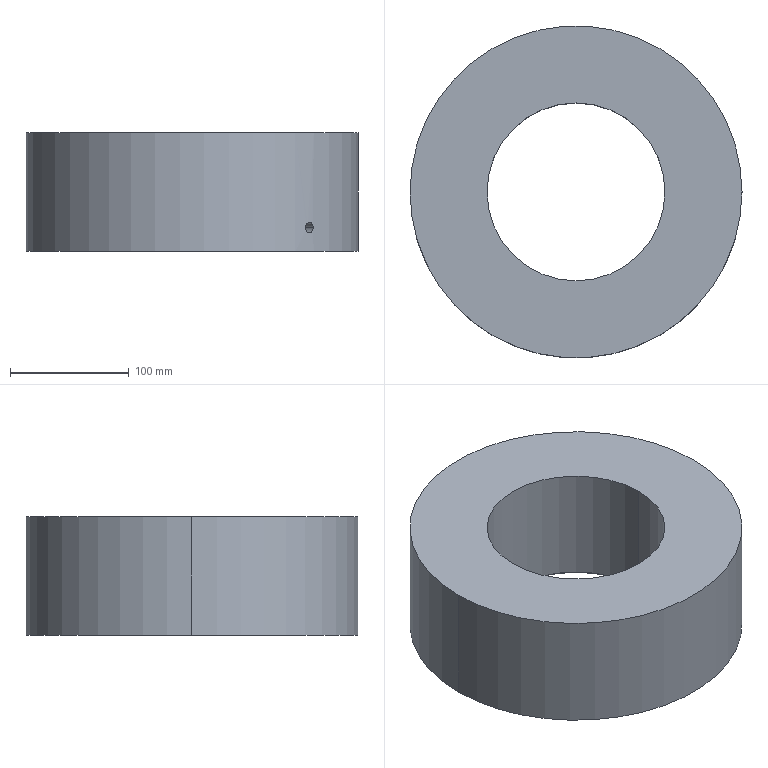Component | SolidWorks | JF21-80.1-1-3(_)-1-SOLID27-1 | 1 solid | 14 faces | box 280 x 280 x 100 mm | volume 4386913 mm3 | cylinder 8 | cone 4 | plane 2 | commonest cylinder face diameters 9 x2 7.5 x2 150 x2 280 x2
STEP:
#1=COLOUR_RGB('',0.7922,0.8196,0.9333);
#2=FILL_AREA_STYLE_COLOUR('',#1);
#3=FILL_AREA_STYLE('',(#2));
#4=SURFACE_STYLE_FILL_AREA(#3);
#5=SURFACE_SIDE_STYLE('',(#4));
#6=SURFACE_STYLE_USAGE(.BOTH.,#5);
#7=PRESENTATION_STYLE_ASSIGNMENT((#6));
#8=CARTESIAN_POINT('',(2.953,0.,7.323));
#9=VERTEX_POINT('',#8);
#10=CARTESIAN_POINT('',(-2.953,0.,7.323));
#11=VERTEX_POINT('',#10);
#12=CARTESIAN_POINT('',(0.,0.,7.323));
#13=DIRECTION('',(0.,0.,-1.));
#14=DIRECTION('',(1.,0.,0.));
#15=AXIS2_PLACEMENT_3D('',#12,#13,#14);
#16=CIRCLE('',#15,2.953);
#17=EDGE_CURVE('',#9,#11,#16,.T.);
#18=ORIENTED_EDGE('',*,*,#17,.F.);
#19=CARTESIAN_POINT('',(2.992,0.,7.283));
#20=VERTEX_POINT('',#19);
#21=CARTESIAN_POINT('',(2.992,0.,7.283));
#22=DIRECTION('',(-0.7071,-0.,0.7071));
#23=VECTOR('',#22,39.37);
#24=LINE('',#21,#23);
#25=EDGE_CURVE('',#20,#9,#24,.T.);
#26=ORIENTED_EDGE('',*,*,#25,.F.);
#27=CARTESIAN_POINT('',(-2.992,0.,7.283));
#28=VERTEX_POINT('',#27);
#29=CARTESIAN_POINT('',(0.,0.,7.283));
#30=DIRECTION('',(0.,0.,1.));
#31=DIRECTION('',(1.,0.,0.));
#32=AXIS2_PLACEMENT_3D('',#29,#30,#31);
#33=CIRCLE('',#32,2.992);
#34=EDGE_CURVE('',#28,#20,#33,.T.);
#35=ORIENTED_EDGE('',*,*,#34,.F.);
#36=CARTESIAN_POINT('',(-2.992,0.,7.283));
#37=DIRECTION('',(0.7071,0.,0.7071));
#38=VECTOR('',#37,39.37);
#39=LINE('',#36,#38);
#40=EDGE_CURVE('',#28,#11,#39,.T.);
#41=ORIENTED_EDGE('',*,*,#40,.T.);
#42=EDGE_LOOP('',(#18,#26,#35,#41));
#43=FACE_OUTER_BOUND('',#42,.T.);
#44=CARTESIAN_POINT('',(0.,0.,7.283));
#45=DIRECTION('',(0.,0.,-1.));
#46=DIRECTION('',(1.,0.,0.));
#47=AXIS2_PLACEMENT_3D('',#44,#45,#46);
#48=CONICAL_SURFACE('',#47,2.992,0.7854);
#49=ADVANCED_FACE('',(#43),#48,.F.);
#50=CARTESIAN_POINT('',(3.271,-3.522,8.071));
#51=VERTEX_POINT('',#50);
#52=CARTESIAN_POINT('',(3.522,-3.271,8.071));
#53=VERTEX_POINT('',#52);
#54=CARTESIAN_POINT('',(3.396,-3.396,8.071));
#55=DIRECTION('',(0.7071,-0.7071,0.));
#56=DIRECTION('',(0.7071,0.7071,0.));
#57=AXIS2_PLACEMENT_3D('',#54,#55,#56);
#58=CIRCLE('',#57,0.1772);
#59=EDGE_CURVE('',#51,#53,#58,.T.);
#60=ORIENTED_EDGE('',*,*,#59,.F.);
#61=CARTESIAN_POINT('',(3.77,-4.021,8.071));
#62=VERTEX_POINT('',#61);
#63=CARTESIAN_POINT('',(3.772,-4.023,8.071));
#64=DIRECTION('',(0.7071,-0.7071,0.));
#65=VECTOR('',#64,39.37);
#66=LINE('',#63,#65);
#67=EDGE_CURVE('',#51,#62,#66,.T.);
#68=ORIENTED_EDGE('',*,*,#67,.T.);
#69=CARTESIAN_POINT('',(4.021,-3.77,8.071));
#70=VERTEX_POINT('',#69);
#71=CARTESIAN_POINT('',(3.77,-4.021,8.071));
#72=CARTESIAN_POINT('',(3.77,-4.021,8.059));
#73=CARTESIAN_POINT('',(3.771,-4.02,8.048));
#74=CARTESIAN_POINT('',(3.774,-4.017,8.025));
#75=CARTESIAN_POINT('',(3.777,-4.014,8.014));
#76=CARTESIAN_POINT('',(3.783,-4.008,7.992));
#77=CARTESIAN_POINT('',(3.787,-4.005,7.982));
#78=CARTESIAN_POINT('',(3.797,-3.996,7.963));
#79=CARTESIAN_POINT('',(3.802,-3.991,7.954));
#80=CARTESIAN_POINT('',(3.814,-3.979,7.937));
#81=CARTESIAN_POINT('',(3.82,-3.973,7.93));
#82=CARTESIAN_POINT('',(3.834,-3.96,7.917));
#83=CARTESIAN_POINT('',(3.842,-3.953,7.912));
#84=CARTESIAN_POINT('',(3.857,-3.938,7.903));
#85=CARTESIAN_POINT('',(3.865,-3.93,7.899));
#86=CARTESIAN_POINT('',(3.881,-3.914,7.895));
#87=CARTESIAN_POINT('',(3.889,-3.906,7.894));
#88=CARTESIAN_POINT('',(3.906,-3.889,7.894));
#89=CARTESIAN_POINT('',(3.914,-3.881,7.895));
#90=CARTESIAN_POINT('',(3.93,-3.865,7.899));
#91=CARTESIAN_POINT('',(3.937,-3.857,7.903));
#92=CARTESIAN_POINT('',(3.952,-3.842,7.912));
#93=CARTESIAN_POINT('',(3.96,-3.834,7.917));
#94=CARTESIAN_POINT('',(3.973,-3.82,7.93));
#95=CARTESIAN_POINT('',(3.979,-3.814,7.937));
#96=CARTESIAN_POINT('',(3.991,-3.802,7.954));
#97=CARTESIAN_POINT('',(3.996,-3.797,7.963));
#98=CARTESIAN_POINT('',(4.005,-3.787,7.982));
#99=CARTESIAN_POINT('',(4.008,-3.783,7.992));
#100=CARTESIAN_POINT('',(4.014,-3.777,8.014));
#101=CARTESIAN_POINT('',(4.017,-3.774,8.025));
#102=CARTESIAN_POINT('',(4.02,-3.771,8.047));
#103=CARTESIAN_POINT('',(4.021,-3.77,8.059));
#104=CARTESIAN_POINT('',(4.021,-3.77,8.071));
#105=B_SPLINE_CURVE_WITH_KNOTS('',3,(#71,#72,#73,#74,#75,#76,#77,#78,#79,#80,#81,#82,#83,#84,#85,#86,#87,#88,#89,#90,#91,#92,#93,#94,#95,#96,#97,#98,#99,#100,#101,#102,#103,#104),.UNSPECIFIED.,.F.,.F.,(4,2,2,2,2,2,2,2,2,2,2,2,2,2,2,2,4),(0.,0.0008792,0.001758,0.002638,0.003517,0.004396,0.005275,0.006154,0.007034,0.007913,0.008792,0.009671,0.01055,0.01143,0.01231,0.01319,0.01407),.UNSPECIFIED.);
#106=EDGE_CURVE('',#62,#70,#105,.T.);
#107=ORIENTED_EDGE('',*,*,#106,.T.);
#108=CARTESIAN_POINT('',(4.023,-3.772,8.071));
#109=DIRECTION('',(0.7071,-0.7071,0.));
#110=VECTOR('',#109,39.37);
#111=LINE('',#108,#110);
#112=EDGE_CURVE('',#53,#70,#111,.T.);
#113=ORIENTED_EDGE('',*,*,#112,.F.);
#114=EDGE_LOOP('',(#60,#68,#107,#113));
#115=FACE_OUTER_BOUND('',#114,.T.);
#116=CARTESIAN_POINT('',(3.897,-3.897,8.071));
#117=DIRECTION('',(0.7071,-0.7071,0.));
#118=DIRECTION('',(-0.7071,-0.7071,0.));
#119=AXIS2_PLACEMENT_3D('',#116,#117,#118);
#120=CYLINDRICAL_SURFACE('',#119,0.1772);
#121=ADVANCED_FACE('',(#115),#120,.F.);
#122=CARTESIAN_POINT('',(3.279,-3.488,8.071));
#123=VERTEX_POINT('',#122);
#124=CARTESIAN_POINT('',(3.488,-3.279,8.071));
#125=VERTEX_POINT('',#124);
#126=CARTESIAN_POINT('',(3.384,-3.384,8.071));
#127=DIRECTION('',(0.7071,-0.7071,0.));
#128=DIRECTION('',(0.7071,0.7071,0.));
#129=AXIS2_PLACEMENT_3D('',#126,#127,#128);
#130=CIRCLE('',#129,0.1476);
#131=EDGE_CURVE('',#123,#125,#130,.T.);
#132=ORIENTED_EDGE('',*,*,#131,.F.);
#133=CARTESIAN_POINT('',(3.271,-3.522,8.071));
#134=DIRECTION('',(-0.2419,-0.9703,0.));
#135=VECTOR('',#134,39.37);
#136=LINE('',#133,#135);
#137=EDGE_CURVE('',#123,#51,#136,.T.);
#138=ORIENTED_EDGE('',*,*,#137,.T.);
#139=ORIENTED_EDGE('',*,*,#59,.T.);
#140=CARTESIAN_POINT('',(3.522,-3.271,8.071));
#141=DIRECTION('',(0.9703,0.2419,0.));
#142=VECTOR('',#141,39.37);
#143=LINE('',#140,#142);
#144=EDGE_CURVE('',#125,#53,#143,.T.);
#145=ORIENTED_EDGE('',*,*,#144,.F.);
#146=EDGE_LOOP('',(#132,#138,#139,#145));
#147=FACE_OUTER_BOUND('',#146,.T.);
#148=CARTESIAN_POINT('',(3.396,-3.396,8.071));
#149=DIRECTION('',(0.7071,-0.7071,0.));
#150=DIRECTION('',(-0.7071,-0.7071,0.));
#151=AXIS2_PLACEMENT_3D('',#148,#149,#150);
#152=CONICAL_SURFACE('',#151,0.1772,1.03);
#153=ADVANCED_FACE('',(#147),#152,.F.);
#154=CARTESIAN_POINT('',(1.981,-2.19,8.071));
#155=VERTEX_POINT('',#154);
#156=CARTESIAN_POINT('',(2.19,-1.981,8.071));
#157=VERTEX_POINT('',#156);
#158=CARTESIAN_POINT('',(1.981,-2.19,8.071));
#159=CARTESIAN_POINT('',(1.981,-2.19,8.061));
#160=CARTESIAN_POINT('',(1.982,-2.189,8.052));
#161=CARTESIAN_POINT('',(1.984,-2.187,8.033));
#162=CARTESIAN_POINT('',(1.987,-2.185,8.023));
#163=CARTESIAN_POINT('',(1.992,-2.18,8.005));
#164=CARTESIAN_POINT('',(1.995,-2.177,7.997));
#165=CARTESIAN_POINT('',(2.003,-2.169,7.981));
#166=CARTESIAN_POINT('',(2.008,-2.165,7.973));
#167=CARTESIAN_POINT('',(2.018,-2.156,7.96));
#168=CARTESIAN_POINT('',(2.023,-2.151,7.954));
#169=CARTESIAN_POINT('',(2.035,-2.14,7.943));
#170=CARTESIAN_POINT('',(2.041,-2.134,7.938));
#171=CARTESIAN_POINT('',(2.054,-2.121,7.931));
#172=CARTESIAN_POINT('',(2.061,-2.115,7.928));
#173=CARTESIAN_POINT('',(2.074,-2.102,7.924));
#174=CARTESIAN_POINT('',(2.081,-2.095,7.923));
#175=CARTESIAN_POINT('',(2.095,-2.081,7.923));
#176=CARTESIAN_POINT('',(2.102,-2.074,7.924));
#177=CARTESIAN_POINT('',(2.115,-2.061,7.928));
#178=CARTESIAN_POINT('',(2.121,-2.054,7.931));
#179=CARTESIAN_POINT('',(2.134,-2.041,7.938));
#180=CARTESIAN_POINT('',(2.14,-2.035,7.943));
#181=CARTESIAN_POINT('',(2.151,-2.023,7.953));
#182=CARTESIAN_POINT('',(2.156,-2.018,7.96));
#183=CARTESIAN_POINT('',(2.165,-2.008,7.973));
#184=CARTESIAN_POINT('',(2.169,-2.003,7.981));
#185=CARTESIAN_POINT('',(2.176,-1.995,7.997));
#186=CARTESIAN_POINT('',(2.18,-1.992,8.005));
#187=CARTESIAN_POINT('',(2.185,-1.987,8.023));
#188=CARTESIAN_POINT('',(2.186,-1.984,8.032));
#189=CARTESIAN_POINT('',(2.189,-1.982,8.051));
#190=CARTESIAN_POINT('',(2.19,-1.981,8.061));
#191=CARTESIAN_POINT('',(2.19,-1.981,8.071));
#192=B_SPLINE_CURVE_WITH_KNOTS('',3,(#158,#159,#160,#161,#162,#163,#164,#165,#166,#167,#168,#169,#170,#171,#172,#173,#174,#175,#176,#177,#178,#179,#180,#181,#182,#183,#184,#185,#186,#187,#188,#189,#190,#191),.UNSPECIFIED.,.F.,.F.,(4,2,2,2,2,2,2,2,2,2,2,2,2,2,2,2,4),(0.,0.0007327,0.001465,0.002198,0.002931,0.003664,0.004396,0.005129,0.005862,0.006595,0.007327,0.00806,0.008793,0.009525,0.01026,0.01099,0.01172),.UNSPECIFIED.);
#193=EDGE_CURVE('',#155,#157,#192,.T.);
#194=ORIENTED_EDGE('',*,*,#193,.F.);
#195=CARTESIAN_POINT('',(3.793,-4.002,8.071));
#196=DIRECTION('',(0.7071,-0.7071,0.));
#197=VECTOR('',#196,39.37);
#198=LINE('',#195,#197);
#199=EDGE_CURVE('',#155,#123,#198,.T.);
#200=ORIENTED_EDGE('',*,*,#199,.T.);
#201=ORIENTED_EDGE('',*,*,#131,.T.);
#202=CARTESIAN_POINT('',(4.002,-3.793,8.071));
#203=DIRECTION('',(0.7071,-0.7071,0.));
#204=VECTOR('',#203,39.37);
#205=LINE('',#202,#204);
#206=EDGE_CURVE('',#157,#125,#205,.T.);
#207=ORIENTED_EDGE('',*,*,#206,.F.);
#208=EDGE_LOOP('',(#194,#200,#201,#207));
#209=FACE_OUTER_BOUND('',#208,.T.);
#210=CARTESIAN_POINT('',(3.897,-3.897,8.071));
#211=DIRECTION('',(0.7071,-0.7071,0.));
#212=DIRECTION('',(-0.7071,-0.7071,0.));
#213=AXIS2_PLACEMENT_3D('',#210,#211,#212);
#214=CYLINDRICAL_SURFACE('',#213,0.1476);
#215=ADVANCED_FACE('',(#209),#214,.F.);
#216=CARTESIAN_POINT('',(2.19,-1.981,8.071));
#217=CARTESIAN_POINT('',(2.19,-1.981,8.081));
#218=CARTESIAN_POINT('',(2.189,-1.982,8.09));
#219=CARTESIAN_POINT('',(2.187,-1.984,8.109));
#220=CARTESIAN_POINT('',(2.185,-1.987,8.118));
#221=CARTESIAN_POINT('',(2.18,-1.992,8.136));
#222=CARTESIAN_POINT('',(2.177,-1.995,8.145));
#223=CARTESIAN_POINT('',(2.169,-2.003,8.161));
#224=CARTESIAN_POINT('',(2.165,-2.008,8.168));
#225=CARTESIAN_POINT('',(2.156,-2.018,8.182));
#226=CARTESIAN_POINT('',(2.151,-2.023,8.188));
#227=CARTESIAN_POINT('',(2.14,-2.035,8.199));
#228=CARTESIAN_POINT('',(2.134,-2.041,8.204));
#229=CARTESIAN_POINT('',(2.121,-2.054,8.211));
#230=CARTESIAN_POINT('',(2.115,-2.061,8.214));
#231=CARTESIAN_POINT('',(2.102,-2.074,8.218));
#232=CARTESIAN_POINT('',(2.095,-2.081,8.218));
#233=CARTESIAN_POINT('',(2.081,-2.095,8.219));
#234=CARTESIAN_POINT('',(2.074,-2.102,8.218));
#235=CARTESIAN_POINT('',(2.061,-2.115,8.214));
#236=CARTESIAN_POINT('',(2.054,-2.121,8.211));
#237=CARTESIAN_POINT('',(2.041,-2.134,8.204));
#238=CARTESIAN_POINT('',(2.035,-2.14,8.199));
#239=CARTESIAN_POINT('',(2.023,-2.151,8.188));
#240=CARTESIAN_POINT('',(2.018,-2.156,8.182));
#241=CARTESIAN_POINT('',(2.008,-2.165,8.168));
#242=CARTESIAN_POINT('',(2.003,-2.169,8.161));
#243=CARTESIAN_POINT('',(1.995,-2.176,8.145));
#244=CARTESIAN_POINT('',(1.992,-2.18,8.136));
#245=CARTESIAN_POINT('',(1.987,-2.185,8.118));
#246=CARTESIAN_POINT('',(1.984,-2.186,8.109));
#247=CARTESIAN_POINT('',(1.982,-2.189,8.09));
#248=CARTESIAN_POINT('',(1.981,-2.19,8.081));
#249=CARTESIAN_POINT('',(1.981,-2.19,8.071));
#250=B_SPLINE_CURVE_WITH_KNOTS('',3,(#216,#217,#218,#219,#220,#221,#222,#223,#224,#225,#226,#227,#228,#229,#230,#231,#232,#233,#234,#235,#236,#237,#238,#239,#240,#241,#242,#243,#244,#245,#246,#247,#248,#249),.UNSPECIFIED.,.F.,.F.,(4,2,2,2,2,2,2,2,2,2,2,2,2,2,2,2,4),(0.,0.0007327,0.001465,0.002198,0.002931,0.003664,0.004396,0.005129,0.005862,0.006595,0.007327,0.00806,0.008793,0.009525,0.01026,0.01099,0.01172),.UNSPECIFIED.);
#251=EDGE_CURVE('',#157,#155,#250,.T.);
#252=ORIENTED_EDGE('',*,*,#251,.T.);
#253=ORIENTED_EDGE('',*,*,#193,.T.);
#254=EDGE_LOOP('',(#252,#253));
#255=FACE_BOUND('',#254,.T.);
#256=ORIENTED_EDGE('',*,*,#17,.T.);
#257=CARTESIAN_POINT('',(-2.953,0.,11.22));
#258=VERTEX_POINT('',#257);
#259=CARTESIAN_POINT('',(-2.953,0.,7.283));
#260=DIRECTION('',(0.,0.,1.));
#261=VECTOR('',#260,39.37);
#262=LINE('',#259,#261);
#263=EDGE_CURVE('',#11,#258,#262,.T.);
#264=ORIENTED_EDGE('',*,*,#263,.T.);
#265=CARTESIAN_POINT('',(2.953,0.,11.22));
#266=VERTEX_POINT('',#265);
#267=CARTESIAN_POINT('',(0.,0.,11.22));
#268=DIRECTION('',(0.,0.,1.));
#269=DIRECTION('',(1.,0.,0.));
#270=AXIS2_PLACEMENT_3D('',#267,#268,#269);
#271=CIRCLE('',#270,2.953);
#272=EDGE_CURVE('',#258,#266,#271,.T.);
#273=ORIENTED_EDGE('',*,*,#272,.T.);
#274=CARTESIAN_POINT('',(2.953,0.,7.283));
#275=DIRECTION('',(0.,0.,1.));
#276=VECTOR('',#275,39.37);
#277=LINE('',#274,#276);
#278=EDGE_CURVE('',#9,#266,#277,.T.);
#279=ORIENTED_EDGE('',*,*,#278,.F.);
#280=EDGE_LOOP('',(#256,#264,#273,#279));
#281=FACE_OUTER_BOUND('',#280,.T.);
#282=CARTESIAN_POINT('',(0.,0.,7.283));
#283=DIRECTION('',(0.,0.,1.));
#284=DIRECTION('',(-1.,0.,0.));
#285=AXIS2_PLACEMENT_3D('',#282,#283,#284);
#286=CYLINDRICAL_SURFACE('',#285,2.953);
#287=ADVANCED_FACE('',(#255,#281),#286,.F.);
#288=CARTESIAN_POINT('',(5.512,0.,7.283));
#289=VERTEX_POINT('',#288);
#290=CARTESIAN_POINT('',(-5.512,0.,7.283));
#291=VERTEX_POINT('',#290);
#292=CARTESIAN_POINT('',(0.,0.,7.283));
#293=DIRECTION('',(0.,0.,1.));
#294=DIRECTION('',(1.,0.,0.));
#295=AXIS2_PLACEMENT_3D('',#292,#293,#294);
#296=CIRCLE('',#295,5.512);
#297=EDGE_CURVE('',#289,#291,#296,.T.);
#298=ORIENTED_EDGE('',*,*,#297,.T.);
#299=CARTESIAN_POINT('',(-5.512,0.,11.22));
#300=VERTEX_POINT('',#299);
#301=CARTESIAN_POINT('',(-5.512,0.,7.283));
#302=DIRECTION('',(0.,0.,1.));
#303=VECTOR('',#302,39.37);
#304=LINE('',#301,#303);
#305=EDGE_CURVE('',#291,#300,#304,.T.);
#306=ORIENTED_EDGE('',*,*,#305,.T.);
#307=CARTESIAN_POINT('',(5.512,0.,11.22));
#308=VERTEX_POINT('',#307);
#309=CARTESIAN_POINT('',(0.,0.,11.22));
#310=DIRECTION('',(0.,0.,1.));
#311=DIRECTION('',(1.,0.,0.));
#312=AXIS2_PLACEMENT_3D('',#309,#310,#311);
#313=CIRCLE('',#312,5.512);
#314=EDGE_CURVE('',#308,#300,#313,.T.);
#315=ORIENTED_EDGE('',*,*,#314,.F.);
#316=CARTESIAN_POINT('',(5.512,0.,7.283));
#317=DIRECTION('',(0.,0.,1.));
#318=VECTOR('',#317,39.37);
#319=LINE('',#316,#318);
#320=EDGE_CURVE('',#289,#308,#319,.T.);
#321=ORIENTED_EDGE('',*,*,#320,.F.);
#322=EDGE_LOOP('',(#298,#306,#315,#321));
#323=FACE_OUTER_BOUND('',#322,.T.);
#324=CARTESIAN_POINT('',(0.,0.,7.283));
#325=DIRECTION('',(0.,0.,1.));
#326=DIRECTION('',(-1.,0.,0.));
#327=AXIS2_PLACEMENT_3D('',#324,#325,#326);
#328=CYLINDRICAL_SURFACE('',#327,5.512);
#329=ADVANCED_FACE('',(#323),#328,.T.);
#330=ORIENTED_EDGE('',*,*,#305,.F.);
#331=CARTESIAN_POINT('',(0.,0.,7.283));
#332=DIRECTION('',(0.,0.,1.));
#333=DIRECTION('',(1.,0.,0.));
#334=AXIS2_PLACEMENT_3D('',#331,#332,#333);
#335=CIRCLE('',#334,5.512);
#336=EDGE_CURVE('',#291,#289,#335,.T.);
#337=ORIENTED_EDGE('',*,*,#336,.T.);
#338=ORIENTED_EDGE('',*,*,#320,.T.);
#339=CARTESIAN_POINT('',(0.,0.,11.22));
#340=DIRECTION('',(0.,0.,1.));
#341=DIRECTION('',(1.,0.,0.));
#342=AXIS2_PLACEMENT_3D('',#339,#340,#341);
#343=CIRCLE('',#342,5.512);
#344=EDGE_CURVE('',#300,#308,#343,.T.);
#345=ORIENTED_EDGE('',*,*,#344,.F.);
#346=EDGE_LOOP('',(#330,#337,#338,#345));
#347=FACE_OUTER_BOUND('',#346,.T.);
#348=CARTESIAN_POINT('',(4.021,-3.77,8.071));
#349=CARTESIAN_POINT('',(4.021,-3.77,8.083));
#350=CARTESIAN_POINT('',(4.02,-3.771,8.094));
#351=CARTESIAN_POINT('',(4.017,-3.774,8.117));
#352=CARTESIAN_POINT('',(4.014,-3.777,8.128));
#353=CARTESIAN_POINT('',(4.008,-3.783,8.149));
#354=CARTESIAN_POINT('',(4.005,-3.787,8.16));
#355=CARTESIAN_POINT('',(3.996,-3.797,8.179));
#356=CARTESIAN_POINT('',(3.991,-3.802,8.188));
#357=CARTESIAN_POINT('',(3.979,-3.814,8.204));
#358=CARTESIAN_POINT('',(3.973,-3.82,8.212));
#359=CARTESIAN_POINT('',(3.96,-3.834,8.225));
#360=CARTESIAN_POINT('',(3.953,-3.842,8.23));
#361=CARTESIAN_POINT('',(3.938,-3.857,8.239));
#362=CARTESIAN_POINT('',(3.93,-3.865,8.242));
#363=CARTESIAN_POINT('',(3.914,-3.881,8.247));
#364=CARTESIAN_POINT('',(3.906,-3.889,8.248));
#365=CARTESIAN_POINT('',(3.889,-3.906,8.248));
#366=CARTESIAN_POINT('',(3.881,-3.914,8.247));
#367=CARTESIAN_POINT('',(3.865,-3.93,8.242));
#368=CARTESIAN_POINT('',(3.857,-3.937,8.239));
#369=CARTESIAN_POINT('',(3.842,-3.952,8.23));
#370=CARTESIAN_POINT('',(3.834,-3.96,8.225));
#371=CARTESIAN_POINT('',(3.82,-3.973,8.212));
#372=CARTESIAN_POINT('',(3.814,-3.979,8.204));
#373=CARTESIAN_POINT('',(3.802,-3.991,8.188));
#374=CARTESIAN_POINT('',(3.797,-3.996,8.179));
#375=CARTESIAN_POINT('',(3.787,-4.005,8.16));
#376=CARTESIAN_POINT('',(3.783,-4.008,8.149));
#377=CARTESIAN_POINT('',(3.777,-4.014,8.128));
#378=CARTESIAN_POINT('',(3.774,-4.017,8.117));
#379=CARTESIAN_POINT('',(3.771,-4.02,8.094));
#380=CARTESIAN_POINT('',(3.77,-4.021,8.083));
#381=CARTESIAN_POINT('',(3.77,-4.021,8.071));
#382=B_SPLINE_CURVE_WITH_KNOTS('',3,(#348,#349,#350,#351,#352,#353,#354,#355,#356,#357,#358,#359,#360,#361,#362,#363,#364,#365,#366,#367,#368,#369,#370,#371,#372,#373,#374,#375,#376,#377,#378,#379,#380,#381),.UNSPECIFIED.,.F.,.F.,(4,2,2,2,2,2,2,2,2,2,2,2,2,2,2,2,4),(0.,0.0008792,0.001758,0.002638,0.003517,0.004396,0.005275,0.006154,0.007034,0.007913,0.008792,0.009671,0.01055,0.01143,0.01231,0.01319,0.01407),.UNSPECIFIED.);
#383=EDGE_CURVE('',#70,#62,#382,.T.);
#384=ORIENTED_EDGE('',*,*,#383,.F.);
#385=ORIENTED_EDGE('',*,*,#106,.F.);
#386=EDGE_LOOP('',(#384,#385));
#387=FACE_BOUND('',#386,.T.);
#388=CARTESIAN_POINT('',(0.,0.,7.283));
#389=DIRECTION('',(0.,0.,1.));
#390=DIRECTION('',(-1.,0.,0.));
#391=AXIS2_PLACEMENT_3D('',#388,#389,#390);
#392=CYLINDRICAL_SURFACE('',#391,5.512);
#393=ADVANCED_FACE('',(#347,#387),#392,.T.);
#394=ORIENTED_EDGE('',*,*,#34,.T.);
#395=CARTESIAN_POINT('',(0.,0.,7.283));
#396=DIRECTION('',(0.,0.,1.));
#397=DIRECTION('',(1.,0.,0.));
#398=AXIS2_PLACEMENT_3D('',#395,#396,#397);
#399=CIRCLE('',#398,2.992);
#400=EDGE_CURVE('',#20,#28,#399,.T.);
#401=ORIENTED_EDGE('',*,*,#400,.T.);
#402=EDGE_LOOP('',(#394,#401));
#403=FACE_BOUND('',#402,.T.);
#404=ORIENTED_EDGE('',*,*,#297,.F.);
#405=ORIENTED_EDGE('',*,*,#336,.F.);
#406=EDGE_LOOP('',(#404,#405));
#407=FACE_OUTER_BOUND('',#406,.T.);
#408=CARTESIAN_POINT('',(0.,0.,7.283));
#409=DIRECTION('',(0.,0.,1.));
#410=DIRECTION('',(-1.,0.,0.));
#411=AXIS2_PLACEMENT_3D('',#408,#409,#410);
#412=PLANE('',#411);
#413=ADVANCED_FACE('',(#403,#407),#412,.F.);
#414=CARTESIAN_POINT('',(0.,0.,11.22));
#415=DIRECTION('',(0.,0.,1.));
#416=DIRECTION('',(1.,0.,0.));
#417=AXIS2_PLACEMENT_3D('',#414,#415,#416);
#418=CIRCLE('',#417,2.953);
#419=EDGE_CURVE('',#266,#258,#418,.T.);
#420=ORIENTED_EDGE('',*,*,#419,.F.);
#421=ORIENTED_EDGE('',*,*,#272,.F.);
#422=EDGE_LOOP('',(#420,#421));
#423=FACE_BOUND('',#422,.T.);
#424=ORIENTED_EDGE('',*,*,#314,.T.);
#425=ORIENTED_EDGE('',*,*,#344,.T.);
#426=EDGE_LOOP('',(#424,#425));
#427=FACE_OUTER_BOUND('',#426,.T.);
#428=CARTESIAN_POINT('',(0.,0.,11.22));
#429=DIRECTION('',(0.,0.,1.));
#430=DIRECTION('',(-1.,0.,0.));
#431=AXIS2_PLACEMENT_3D('',#428,#429,#430);
#432=PLANE('',#431);
#433=ADVANCED_FACE('',(#423,#427),#432,.T.);
#434=ORIENTED_EDGE('',*,*,#263,.F.);
#435=CARTESIAN_POINT('',(0.,0.,7.323));
#436=DIRECTION('',(0.,0.,-1.));
#437=DIRECTION('',(1.,0.,0.));
#438=AXIS2_PLACEMENT_3D('',#435,#436,#437);
#439=CIRCLE('',#438,2.953);
#440=EDGE_CURVE('',#11,#9,#439,.T.);
#441=ORIENTED_EDGE('',*,*,#440,.T.);
#442=ORIENTED_EDGE('',*,*,#278,.T.);
#443=ORIENTED_EDGE('',*,*,#419,.T.);
#444=EDGE_LOOP('',(#434,#441,#442,#443));
#445=FACE_OUTER_BOUND('',#444,.T.);
#446=CARTESIAN_POINT('',(0.,0.,7.283));
#447=DIRECTION('',(0.,0.,1.));
#448=DIRECTION('',(-1.,0.,0.));
#449=AXIS2_PLACEMENT_3D('',#446,#447,#448);
#450=CYLINDRICAL_SURFACE('',#449,2.953);
#451=ADVANCED_FACE('',(#445),#450,.F.);
#452=ORIENTED_EDGE('',*,*,#199,.F.);
#453=ORIENTED_EDGE('',*,*,#251,.F.);
#454=ORIENTED_EDGE('',*,*,#206,.T.);
#455=CARTESIAN_POINT('',(3.384,-3.384,8.071));
#456=DIRECTION('',(0.7071,-0.7071,0.));
#457=DIRECTION('',(0.7071,0.7071,0.));
#458=AXIS2_PLACEMENT_3D('',#455,#456,#457);
#459=CIRCLE('',#458,0.1476);
#460=EDGE_CURVE('',#125,#123,#459,.T.);
#461=ORIENTED_EDGE('',*,*,#460,.T.);
#462=EDGE_LOOP('',(#452,#453,#454,#461));
#463=FACE_OUTER_BOUND('',#462,.T.);
#464=CARTESIAN_POINT('',(3.897,-3.897,8.071));
#465=DIRECTION('',(0.7071,-0.7071,0.));
#466=DIRECTION('',(-0.7071,-0.7071,0.));
#467=AXIS2_PLACEMENT_3D('',#464,#465,#466);
#468=CYLINDRICAL_SURFACE('',#467,0.1476);
#469=ADVANCED_FACE('',(#463),#468,.F.);
#470=ORIENTED_EDGE('',*,*,#137,.F.);
#471=ORIENTED_EDGE('',*,*,#460,.F.);
#472=ORIENTED_EDGE('',*,*,#144,.T.);
#473=CARTESIAN_POINT('',(3.396,-3.396,8.071));
#474=DIRECTION('',(0.7071,-0.7071,0.));
#475=DIRECTION('',(0.7071,0.7071,0.));
#476=AXIS2_PLACEMENT_3D('',#473,#474,#475);
#477=CIRCLE('',#476,0.1772);
#478=EDGE_CURVE('',#53,#51,#477,.T.);
#479=ORIENTED_EDGE('',*,*,#478,.T.);
#480=EDGE_LOOP('',(#470,#471,#472,#479));
#481=FACE_OUTER_BOUND('',#480,.T.);
#482=CARTESIAN_POINT('',(3.396,-3.396,8.071));
#483=DIRECTION('',(0.7071,-0.7071,0.));
#484=DIRECTION('',(-0.7071,-0.7071,0.));
#485=AXIS2_PLACEMENT_3D('',#482,#483,#484);
#486=CONICAL_SURFACE('',#485,0.1772,1.03);
#487=ADVANCED_FACE('',(#481),#486,.F.);
#488=ORIENTED_EDGE('',*,*,#67,.F.);
#489=ORIENTED_EDGE('',*,*,#478,.F.);
#490=ORIENTED_EDGE('',*,*,#112,.T.);
#491=ORIENTED_EDGE('',*,*,#383,.T.);
#492=EDGE_LOOP('',(#488,#489,#490,#491));
#493=FACE_OUTER_BOUND('',#492,.T.);
#494=CARTESIAN_POINT('',(3.897,-3.897,8.071));
#495=DIRECTION('',(0.7071,-0.7071,0.));
#496=DIRECTION('',(-0.7071,-0.7071,0.));
#497=AXIS2_PLACEMENT_3D('',#494,#495,#496);
#498=CYLINDRICAL_SURFACE('',#497,0.1772);
#499=ADVANCED_FACE('',(#493),#498,.F.);
#500=ORIENTED_EDGE('',*,*,#25,.T.);
#501=ORIENTED_EDGE('',*,*,#440,.F.);
#502=ORIENTED_EDGE('',*,*,#40,.F.);
#503=ORIENTED_EDGE('',*,*,#400,.F.);
#504=EDGE_LOOP('',(#500,#501,#502,#503));
#505=FACE_OUTER_BOUND('',#504,.T.);
#506=CARTESIAN_POINT('',(0.,0.,7.283));
#507=DIRECTION('',(0.,0.,-1.));
#508=DIRECTION('',(1.,0.,0.));
#509=AXIS2_PLACEMENT_3D('',#506,#507,#508);
#510=CONICAL_SURFACE('',#509,2.992,0.7854);
#511=ADVANCED_FACE('',(#505),#510,.F.);
#512=CLOSED_SHELL('',(#49,#121,#153,#215,#287,#329,#393,#413,#433,#451,#469,#487,#499,#511));
#513=MANIFOLD_SOLID_BREP('',#512);
#514=STYLED_ITEM('',(#7),#513);
#515=PRESENTATION_LAYER_ASSIGNMENT('','',(#514));
#516=(LENGTH_UNIT()NAMED_UNIT(*)SI_UNIT($,.METRE.));
#517=LENGTH_MEASURE_WITH_UNIT(LENGTH_MEASURE(0.0254),#516);
#518=DIMENSIONAL_EXPONENTS(1.,0.,0.,0.,0.,0.,0.);
#519=(CONVERSION_BASED_UNIT('',#517)LENGTH_UNIT()NAMED_UNIT(#518));
#520=UNCERTAINTY_MEASURE_WITH_UNIT(LENGTH_MEASURE(0.00001),#519,'','');
#521=(NAMED_UNIT(*)PLANE_ANGLE_UNIT()SI_UNIT($,.RADIAN.));
#522=(NAMED_UNIT(*)SI_UNIT($,.STERADIAN.)SOLID_ANGLE_UNIT());
#523=(GEOMETRIC_REPRESENTATION_CONTEXT(3)GLOBAL_UNCERTAINTY_ASSIGNED_CONTEXT((#520))GLOBAL_UNIT_ASSIGNED_CONTEXT((#519,#521,#522))REPRESENTATION_CONTEXT('',''));
#524=MECHANICAL_DESIGN_GEOMETRIC_PRESENTATION_REPRESENTATION('',(#514),#523);
#525=CARTESIAN_POINT('',(0.,0.,0.));
#526=DIRECTION('',(0.,0.,1.));
#527=DIRECTION('',(1.,0.,0.));
#528=AXIS2_PLACEMENT_3D('',#525,#526,#527);
#529=(LENGTH_UNIT()NAMED_UNIT(*)SI_UNIT($,.METRE.));
#530=LENGTH_MEASURE_WITH_UNIT(LENGTH_MEASURE(0.0254),#529);
#531=DIMENSIONAL_EXPONENTS(1.,0.,0.,0.,0.,0.,0.);
#532=(CONVERSION_BASED_UNIT('',#530)LENGTH_UNIT()NAMED_UNIT(#531));
#533=UNCERTAINTY_MEASURE_WITH_UNIT(LENGTH_MEASURE(0.00001),#532,'','');
#534=(NAMED_UNIT(*)PLANE_ANGLE_UNIT()SI_UNIT($,.RADIAN.));
#535=(NAMED_UNIT(*)SI_UNIT($,.STERADIAN.)SOLID_ANGLE_UNIT());
#536=(GEOMETRIC_REPRESENTATION_CONTEXT(3)GLOBAL_UNCERTAINTY_ASSIGNED_CONTEXT((#533))GLOBAL_UNIT_ASSIGNED_CONTEXT((#532,#534,#535))REPRESENTATION_CONTEXT('',''));
#537=ADVANCED_BREP_SHAPE_REPRESENTATION('',(#513,#528),#536);